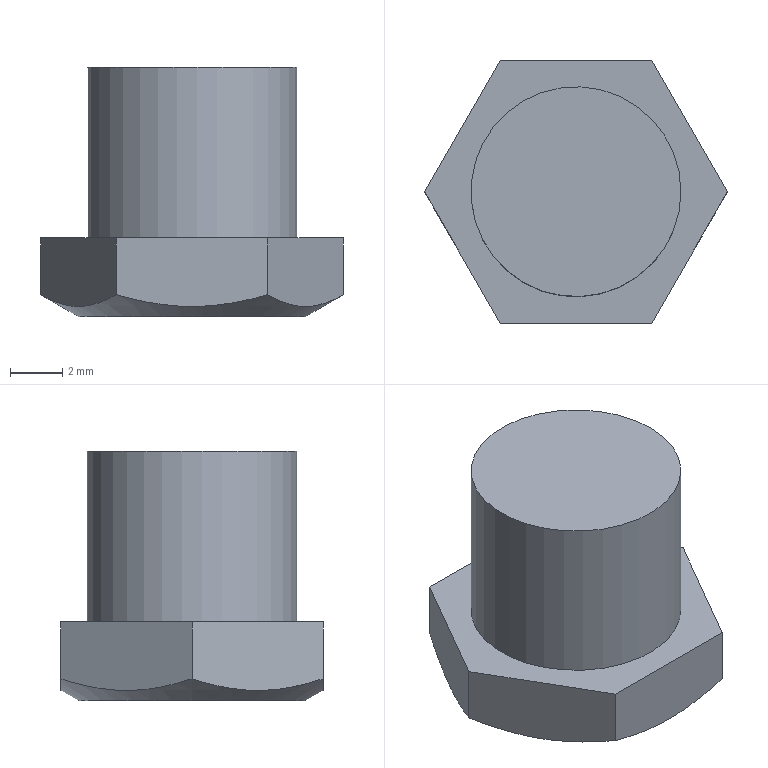Component | NX | BOLT_2 | 1 solid | 11 faces | box 11.55 x 10 x 9.5 mm | volume 578 mm3 | plane 9 | cylinder 1 | cone 1 | commonest cylinder face diameters 8 x1
STEP:
#1=CARTESIAN_POINT('',(0.,0.,0.));
#2=DIRECTION('',(0.,0.,1.));
#3=DIRECTION('',(1.,0.,0.));
#4=AXIS2_PLACEMENT_3D('',#1,#2,#3);
#5=CARTESIAN_POINT('',(-107.5,59.,11.));
#6=VERTEX_POINT('',#5);
#7=CARTESIAN_POINT('',(-111.5,59.,11.));
#8=DIRECTION('',(0.,0.,-1.));
#9=DIRECTION('',(1.,0.,0.));
#10=AXIS2_PLACEMENT_3D('',#7,#8,#9);
#11=CIRCLE('',#10,4.);
#12=CARTESIAN_POINT('',(-111.5,59.,11.));
#13=DIRECTION('',(0.,0.,1.));
#14=DIRECTION('',(-1.,0.,0.));
#15=AXIS2_PLACEMENT_3D('',#12,#13,#14);
#16=PLANE('',#15);
#17=CARTESIAN_POINT('',(-4.,0.));
#18=CARTESIAN_POINT('',(-4.,6.928));
#19=CARTESIAN_POINT('',(2.,3.464));
#20=CARTESIAN_POINT('',(8.,0.));
#21=CARTESIAN_POINT('',(2.,-3.464));
#22=CARTESIAN_POINT('',(-4.,-6.928));
#23=CARTESIAN_POINT('',(-4.,0.));
#24=(BOUNDED_CURVE()B_SPLINE_CURVE(2,(#17,#18,#19,#20,#21,#22,#23),.UNSPECIFIED.,.T.,.F.)B_SPLINE_CURVE_WITH_KNOTS((1,2,2,2,2,1),(-2.094,0.,2.094,4.189,6.283,8.378),.UNSPECIFIED.)CURVE()GEOMETRIC_REPRESENTATION_ITEM()RATIONAL_B_SPLINE_CURVE((1.,0.5,1.,0.5,1.,0.5,1.))REPRESENTATION_ITEM(''));
#25=(GEOMETRIC_REPRESENTATION_CONTEXT(2)PARAMETRIC_REPRESENTATION_CONTEXT()REPRESENTATION_CONTEXT('',''));
#26=DEFINITIONAL_REPRESENTATION('',(#24),#25);
#27=PCURVE('',#16,#26);
#28=CARTESIAN_POINT('',(-111.5,59.,11.));
#29=DIRECTION('',(0.,0.,-1.));
#30=DIRECTION('',(1.,0.,0.));
#31=AXIS2_PLACEMENT_3D('',#28,#29,#30);
#32=CYLINDRICAL_SURFACE('',#31,4.);
#33=CARTESIAN_POINT('',(0.,0.));
#34=DIRECTION('',(1.,0.));
#35=VECTOR('',#34,1.);
#36=LINE('',#33,#35);
#37=(GEOMETRIC_REPRESENTATION_CONTEXT(2)PARAMETRIC_REPRESENTATION_CONTEXT()REPRESENTATION_CONTEXT('',''));
#38=DEFINITIONAL_REPRESENTATION('',(#36),#37);
#39=PCURVE('',#32,#38);
#40=SURFACE_CURVE('',#11,(#27,#39),.PCURVE_S1.);
#41=EDGE_CURVE('',#6,#6,#40,.T.);
#42=ORIENTED_EDGE('',*,*,#41,.F.);
#43=EDGE_LOOP('',(#42));
#44=FACE_BOUND('',#43,.T.);
#45=ADVANCED_FACE('',(#44),#16,.T.);
#46=CARTESIAN_POINT('',(-107.5,59.,4.5));
#47=VERTEX_POINT('',#46);
#48=CARTESIAN_POINT('',(-111.5,59.,4.5));
#49=DIRECTION('',(0.,0.,1.));
#50=DIRECTION('',(1.,0.,0.));
#51=AXIS2_PLACEMENT_3D('',#48,#49,#50);
#52=CIRCLE('',#51,4.);
#53=CARTESIAN_POINT('',(6.283,6.5));
#54=DIRECTION('',(-1.,0.));
#55=VECTOR('',#54,1.);
#56=LINE('',#53,#55);
#57=(GEOMETRIC_REPRESENTATION_CONTEXT(2)PARAMETRIC_REPRESENTATION_CONTEXT()REPRESENTATION_CONTEXT('',''));
#58=DEFINITIONAL_REPRESENTATION('',(#56),#57);
#59=PCURVE('',#32,#58);
#60=CARTESIAN_POINT('',(-111.5,59.,4.5));
#61=DIRECTION('',(0.,0.,1.));
#62=DIRECTION('',(-1.,0.,0.));
#63=AXIS2_PLACEMENT_3D('',#60,#61,#62);
#64=PLANE('',#63);
#65=CARTESIAN_POINT('',(0.,0.));
#66=DIRECTION('',(-1.,0.));
#67=AXIS2_PLACEMENT_2D('',#65,#66);
#68=CIRCLE('',#67,4.);
#69=(GEOMETRIC_REPRESENTATION_CONTEXT(2)PARAMETRIC_REPRESENTATION_CONTEXT()REPRESENTATION_CONTEXT('',''));
#70=DEFINITIONAL_REPRESENTATION('',(#68),#69);
#71=PCURVE('',#64,#70);
#72=SURFACE_CURVE('',#52,(#59,#71),.PCURVE_S1.);
#73=EDGE_CURVE('',#47,#47,#72,.T.);
#74=ORIENTED_EDGE('',*,*,#73,.T.);
#75=CARTESIAN_POINT('',(-107.5,59.,11.));
#76=CARTESIAN_POINT('',(-107.5,59.,4.5));
#77=B_SPLINE_CURVE_WITH_KNOTS('',1,(#75,#76),.UNSPECIFIED.,.F.,.F.,(2,2),(0.,6.5),.PIECEWISE_BEZIER_KNOTS.);
#78=CARTESIAN_POINT('',(0.,0.));
#79=DIRECTION('',(0.,1.));
#80=VECTOR('',#79,1.);
#81=LINE('',#78,#80);
#82=(GEOMETRIC_REPRESENTATION_CONTEXT(2)PARAMETRIC_REPRESENTATION_CONTEXT()REPRESENTATION_CONTEXT('',''));
#83=DEFINITIONAL_REPRESENTATION('',(#81),#82);
#84=PCURVE('',#32,#83);
#85=CARTESIAN_POINT('',(6.283,0.));
#86=DIRECTION('',(0.,1.));
#87=VECTOR('',#86,1.);
#88=LINE('',#85,#87);
#89=(GEOMETRIC_REPRESENTATION_CONTEXT(2)PARAMETRIC_REPRESENTATION_CONTEXT()REPRESENTATION_CONTEXT('',''));
#90=DEFINITIONAL_REPRESENTATION('',(#88),#89);
#91=PCURVE('',#32,#90);
#92=SEAM_CURVE('',#77,(#84,#91),.PCURVE_S1.);
#93=EDGE_CURVE('',#6,#47,#92,.T.);
#94=ORIENTED_EDGE('',*,*,#93,.F.);
#95=ORIENTED_EDGE('',*,*,#41,.T.);
#96=ORIENTED_EDGE('',*,*,#93,.T.);
#97=EDGE_LOOP('',(#74,#94,#95,#96));
#98=FACE_BOUND('',#97,.T.);
#99=ADVANCED_FACE('',(#98),#32,.T.);
#100=CARTESIAN_POINT('',(-105.726,59.,2.333));
#101=VERTEX_POINT('',#100);
#102=CARTESIAN_POINT('',(-108.613,54.,2.333));
#103=VERTEX_POINT('',#102);
#104=CARTESIAN_POINT('',(-105.726,59.,2.333));
#105=CARTESIAN_POINT('',(-106.198,58.184,2.061));
#106=CARTESIAN_POINT('',(-106.676,57.355,1.887));
#107=CARTESIAN_POINT('',(-107.658,55.655,1.886));
#108=CARTESIAN_POINT('',(-108.141,54.817,2.061));
#109=CARTESIAN_POINT('',(-108.613,54.,2.333));
#110=B_SPLINE_CURVE_WITH_KNOTS('',3,(#104,#105,#106,#107,#108,#109),.UNSPECIFIED.,.F.,.F.,(4,2,4),(0.,0.5,1.),.UNSPECIFIED.);
#111=CARTESIAN_POINT('',(-108.613,54.,1.5));
#112=DIRECTION('',(0.866,-0.5,0.));
#113=DIRECTION('',(-0.5,-0.866,0.));
#114=AXIS2_PLACEMENT_3D('',#111,#112,#113);
#115=PLANE('',#114);
#116=CARTESIAN_POINT('',(-5.774,-0.8333));
#117=CARTESIAN_POINT('',(-4.831,-0.5612));
#118=CARTESIAN_POINT('',(-3.874,-0.3874));
#119=CARTESIAN_POINT('',(-1.911,-0.3861));
#120=CARTESIAN_POINT('',(-0.9439,-0.5609));
#121=CARTESIAN_POINT('',(0.,-0.8333));
#122=B_SPLINE_CURVE_WITH_KNOTS('',3,(#116,#117,#118,#119,#120,#121),.UNSPECIFIED.,.F.,.F.,(4,2,4),(0.,0.5,1.),.UNSPECIFIED.);
#123=(GEOMETRIC_REPRESENTATION_CONTEXT(2)PARAMETRIC_REPRESENTATION_CONTEXT()REPRESENTATION_CONTEXT('',''));
#124=DEFINITIONAL_REPRESENTATION('',(#122),#123);
#125=PCURVE('',#115,#124);
#126=CARTESIAN_POINT('',(-111.5,59.,1.5));
#127=DIRECTION('',(0.,0.,1.));
#128=DIRECTION('',(-1.,0.,0.));
#129=AXIS2_PLACEMENT_3D('',#126,#127,#128);
#130=CONICAL_SURFACE('',#129,4.33,1.047);
#131=CARTESIAN_POINT('',(3.142,0.8333));
#132=CARTESIAN_POINT('',(3.129,0.8086));
#133=CARTESIAN_POINT('',(3.102,0.7607));
#134=CARTESIAN_POINT('',(3.061,0.694));
#135=CARTESIAN_POINT('',(3.018,0.6329));
#136=CARTESIAN_POINT('',(2.973,0.5776));
#137=CARTESIAN_POINT('',(2.926,0.5285));
#138=CARTESIAN_POINT('',(2.878,0.4861));
#139=CARTESIAN_POINT('',(2.828,0.4507));
#140=CARTESIAN_POINT('',(2.777,0.4227));
#141=CARTESIAN_POINT('',(2.725,0.4022));
#142=CARTESIAN_POINT('',(2.673,0.3897));
#143=CARTESIAN_POINT('',(2.619,0.3854));
#144=CARTESIAN_POINT('',(2.566,0.3894));
#145=CARTESIAN_POINT('',(2.513,0.4016));
#146=CARTESIAN_POINT('',(2.46,0.4219));
#147=CARTESIAN_POINT('',(2.409,0.4498));
#148=CARTESIAN_POINT('',(2.359,0.4852));
#149=CARTESIAN_POINT('',(2.311,0.5277));
#150=CARTESIAN_POINT('',(2.264,0.5769));
#151=CARTESIAN_POINT('',(2.218,0.6323));
#152=CARTESIAN_POINT('',(2.175,0.6937));
#153=CARTESIAN_POINT('',(2.134,0.7606));
#154=CARTESIAN_POINT('',(2.107,0.8086));
#155=CARTESIAN_POINT('',(2.094,0.8333));
#156=B_SPLINE_CURVE_WITH_KNOTS('',3,(#131,#132,#133,#134,#135,#136,#137,#138,#139,#140,#141,#142,#143,#144,#145,#146,#147,#148,#149,#150,#151,#152,#153,#154,#155),.UNSPECIFIED.,.F.,.F.,(4,1,1,1,1,1,1,1,1,1,1,1,1,1,1,1,1,1,1,1,1,1,4),(0.,0.04545,0.09091,0.1364,0.1818,0.2273,0.2727,0.3182,0.3636,0.4091,0.4545,0.5,0.5455,0.5909,0.6364,0.6818,0.7273,0.7727,0.8182,0.8636,0.9091,0.9545,1.),.QUASI_UNIFORM_KNOTS.);
#157=(GEOMETRIC_REPRESENTATION_CONTEXT(2)PARAMETRIC_REPRESENTATION_CONTEXT()REPRESENTATION_CONTEXT('',''));
#158=DEFINITIONAL_REPRESENTATION('',(#156),#157);
#159=PCURVE('',#130,#158);
#160=SURFACE_CURVE('',#110,(#125,#159),.PCURVE_S1.);
#161=EDGE_CURVE('',#101,#103,#160,.T.);
#162=ORIENTED_EDGE('',*,*,#161,.F.);
#163=CARTESIAN_POINT('',(-105.726,59.,4.5));
#164=VERTEX_POINT('',#163);
#165=CARTESIAN_POINT('',(-105.726,59.,1.5));
#166=DIRECTION('',(0.,0.,1.));
#167=VECTOR('',#166,1.);
#168=LINE('',#165,#167);
#169=CARTESIAN_POINT('',(-5.774,0.));
#170=DIRECTION('',(0.,-1.));
#171=VECTOR('',#170,1.);
#172=LINE('',#169,#171);
#173=(GEOMETRIC_REPRESENTATION_CONTEXT(2)PARAMETRIC_REPRESENTATION_CONTEXT()REPRESENTATION_CONTEXT('',''));
#174=DEFINITIONAL_REPRESENTATION('',(#172),#173);
#175=PCURVE('',#115,#174);
#176=CARTESIAN_POINT('',(-105.726,59.,1.5));
#177=DIRECTION('',(0.866,0.5,0.));
#178=DIRECTION('',(0.5,-0.866,0.));
#179=AXIS2_PLACEMENT_3D('',#176,#177,#178);
#180=PLANE('',#179);
#181=CARTESIAN_POINT('',(0.,0.));
#182=DIRECTION('',(0.,-1.));
#183=VECTOR('',#182,1.);
#184=LINE('',#181,#183);
#185=(GEOMETRIC_REPRESENTATION_CONTEXT(2)PARAMETRIC_REPRESENTATION_CONTEXT()REPRESENTATION_CONTEXT('',''));
#186=DEFINITIONAL_REPRESENTATION('',(#184),#185);
#187=PCURVE('',#180,#186);
#188=SURFACE_CURVE('',#168,(#175,#187),.PCURVE_S1.);
#189=EDGE_CURVE('',#101,#164,#188,.T.);
#190=ORIENTED_EDGE('',*,*,#189,.T.);
#191=CARTESIAN_POINT('',(-108.613,54.,4.5));
#192=VERTEX_POINT('',#191);
#193=CARTESIAN_POINT('',(-108.613,54.,4.5));
#194=DIRECTION('',(0.5,0.866,0.));
#195=VECTOR('',#194,1.);
#196=LINE('',#193,#195);
#197=CARTESIAN_POINT('',(0.,-3.));
#198=DIRECTION('',(-1.,0.));
#199=VECTOR('',#198,1.);
#200=LINE('',#197,#199);
#201=(GEOMETRIC_REPRESENTATION_CONTEXT(2)PARAMETRIC_REPRESENTATION_CONTEXT()REPRESENTATION_CONTEXT('',''));
#202=DEFINITIONAL_REPRESENTATION('',(#200),#201);
#203=PCURVE('',#115,#202);
#204=CARTESIAN_POINT('',(-2.887,5.));
#205=DIRECTION('',(-0.5,-0.866));
#206=VECTOR('',#205,1.);
#207=LINE('',#204,#206);
#208=(GEOMETRIC_REPRESENTATION_CONTEXT(2)PARAMETRIC_REPRESENTATION_CONTEXT()REPRESENTATION_CONTEXT('',''));
#209=DEFINITIONAL_REPRESENTATION('',(#207),#208);
#210=PCURVE('',#64,#209);
#211=SURFACE_CURVE('',#196,(#203,#210),.PCURVE_S1.);
#212=EDGE_CURVE('',#192,#164,#211,.T.);
#213=ORIENTED_EDGE('',*,*,#212,.F.);
#214=CARTESIAN_POINT('',(-108.613,54.,1.5));
#215=DIRECTION('',(0.,0.,1.));
#216=VECTOR('',#215,1.);
#217=LINE('',#214,#216);
#218=CARTESIAN_POINT('',(0.,0.));
#219=DIRECTION('',(0.,-1.));
#220=VECTOR('',#219,1.);
#221=LINE('',#218,#220);
#222=(GEOMETRIC_REPRESENTATION_CONTEXT(2)PARAMETRIC_REPRESENTATION_CONTEXT()REPRESENTATION_CONTEXT('',''));
#223=DEFINITIONAL_REPRESENTATION('',(#221),#222);
#224=PCURVE('',#115,#223);
#225=CARTESIAN_POINT('',(-114.387,54.,1.5));
#226=DIRECTION('',(0.,-1.,0.));
#227=DIRECTION('',(-1.,-0.,0.));
#228=AXIS2_PLACEMENT_3D('',#225,#226,#227);
#229=PLANE('',#228);
#230=CARTESIAN_POINT('',(-5.774,0.));
#231=DIRECTION('',(0.,-1.));
#232=VECTOR('',#231,1.);
#233=LINE('',#230,#232);
#234=(GEOMETRIC_REPRESENTATION_CONTEXT(2)PARAMETRIC_REPRESENTATION_CONTEXT()REPRESENTATION_CONTEXT('',''));
#235=DEFINITIONAL_REPRESENTATION('',(#233),#234);
#236=PCURVE('',#229,#235);
#237=SURFACE_CURVE('',#217,(#224,#236),.PCURVE_S1.);
#238=EDGE_CURVE('',#103,#192,#237,.T.);
#239=ORIENTED_EDGE('',*,*,#238,.F.);
#240=EDGE_LOOP('',(#162,#190,#213,#239));
#241=FACE_BOUND('',#240,.T.);
#242=ADVANCED_FACE('',(#241),#115,.T.);
#243=CARTESIAN_POINT('',(-108.613,64.,2.333));
#244=VERTEX_POINT('',#243);
#245=CARTESIAN_POINT('',(-108.613,64.,2.333));
#246=CARTESIAN_POINT('',(-108.142,63.184,2.061));
#247=CARTESIAN_POINT('',(-107.663,62.355,1.887));
#248=CARTESIAN_POINT('',(-106.682,60.655,1.886));
#249=CARTESIAN_POINT('',(-106.198,59.817,2.061));
#250=CARTESIAN_POINT('',(-105.726,59.,2.333));
#251=B_SPLINE_CURVE_WITH_KNOTS('',3,(#245,#246,#247,#248,#249,#250),.UNSPECIFIED.,.F.,.F.,(4,2,4),(0.,0.5,1.),.UNSPECIFIED.);
#252=CARTESIAN_POINT('',(-5.774,-0.8333));
#253=CARTESIAN_POINT('',(-4.831,-0.5612));
#254=CARTESIAN_POINT('',(-3.874,-0.3874));
#255=CARTESIAN_POINT('',(-1.911,-0.3861));
#256=CARTESIAN_POINT('',(-0.9439,-0.5609));
#257=CARTESIAN_POINT('',(0.,-0.8333));
#258=B_SPLINE_CURVE_WITH_KNOTS('',3,(#252,#253,#254,#255,#256,#257),.UNSPECIFIED.,.F.,.F.,(4,2,4),(0.,0.5,1.),.UNSPECIFIED.);
#259=(GEOMETRIC_REPRESENTATION_CONTEXT(2)PARAMETRIC_REPRESENTATION_CONTEXT()REPRESENTATION_CONTEXT('',''));
#260=DEFINITIONAL_REPRESENTATION('',(#258),#259);
#261=PCURVE('',#180,#260);
#262=CARTESIAN_POINT('',(4.189,0.8333));
#263=CARTESIAN_POINT('',(4.176,0.8086));
#264=CARTESIAN_POINT('',(4.15,0.7607));
#265=CARTESIAN_POINT('',(4.108,0.694));
#266=CARTESIAN_POINT('',(4.065,0.6329));
#267=CARTESIAN_POINT('',(4.02,0.5776));
#268=CARTESIAN_POINT('',(3.974,0.5285));
#269=CARTESIAN_POINT('',(3.925,0.4861));
#270=CARTESIAN_POINT('',(3.876,0.4507));
#271=CARTESIAN_POINT('',(3.825,0.4227));
#272=CARTESIAN_POINT('',(3.773,0.4022));
#273=CARTESIAN_POINT('',(3.72,0.3897));
#274=CARTESIAN_POINT('',(3.666,0.3854));
#275=CARTESIAN_POINT('',(3.613,0.3894));
#276=CARTESIAN_POINT('',(3.56,0.4016));
#277=CARTESIAN_POINT('',(3.507,0.4219));
#278=CARTESIAN_POINT('',(3.456,0.4498));
#279=CARTESIAN_POINT('',(3.406,0.4852));
#280=CARTESIAN_POINT('',(3.358,0.5277));
#281=CARTESIAN_POINT('',(3.311,0.5769));
#282=CARTESIAN_POINT('',(3.266,0.6323));
#283=CARTESIAN_POINT('',(3.222,0.6937));
#284=CARTESIAN_POINT('',(3.181,0.7606));
#285=CARTESIAN_POINT('',(3.154,0.8086));
#286=CARTESIAN_POINT('',(3.142,0.8333));
#287=B_SPLINE_CURVE_WITH_KNOTS('',3,(#262,#263,#264,#265,#266,#267,#268,#269,#270,#271,#272,#273,#274,#275,#276,#277,#278,#279,#280,#281,#282,#283,#284,#285,#286),.UNSPECIFIED.,.F.,.F.,(4,1,1,1,1,1,1,1,1,1,1,1,1,1,1,1,1,1,1,1,1,1,4),(0.,0.04545,0.09091,0.1364,0.1818,0.2273,0.2727,0.3182,0.3636,0.4091,0.4545,0.5,0.5455,0.5909,0.6364,0.6818,0.7273,0.7727,0.8182,0.8636,0.9091,0.9545,1.),.QUASI_UNIFORM_KNOTS.);
#288=(GEOMETRIC_REPRESENTATION_CONTEXT(2)PARAMETRIC_REPRESENTATION_CONTEXT()REPRESENTATION_CONTEXT('',''));
#289=DEFINITIONAL_REPRESENTATION('',(#287),#288);
#290=PCURVE('',#130,#289);
#291=SURFACE_CURVE('',#251,(#261,#290),.PCURVE_S1.);
#292=EDGE_CURVE('',#244,#101,#291,.T.);
#293=ORIENTED_EDGE('',*,*,#292,.F.);
#294=CARTESIAN_POINT('',(-108.613,64.,4.5));
#295=VERTEX_POINT('',#294);
#296=CARTESIAN_POINT('',(-108.613,64.,1.5));
#297=DIRECTION('',(0.,0.,1.));
#298=VECTOR('',#297,1.);
#299=LINE('',#296,#298);
#300=CARTESIAN_POINT('',(-5.774,0.));
#301=DIRECTION('',(0.,-1.));
#302=VECTOR('',#301,1.);
#303=LINE('',#300,#302);
#304=(GEOMETRIC_REPRESENTATION_CONTEXT(2)PARAMETRIC_REPRESENTATION_CONTEXT()REPRESENTATION_CONTEXT('',''));
#305=DEFINITIONAL_REPRESENTATION('',(#303),#304);
#306=PCURVE('',#180,#305);
#307=CARTESIAN_POINT('',(-108.613,64.,1.5));
#308=DIRECTION('',(-0.,1.,0.));
#309=DIRECTION('',(1.,0.,0.));
#310=AXIS2_PLACEMENT_3D('',#307,#308,#309);
#311=PLANE('',#310);
#312=CARTESIAN_POINT('',(0.,0.));
#313=DIRECTION('',(0.,-1.));
#314=VECTOR('',#313,1.);
#315=LINE('',#312,#314);
#316=(GEOMETRIC_REPRESENTATION_CONTEXT(2)PARAMETRIC_REPRESENTATION_CONTEXT()REPRESENTATION_CONTEXT('',''));
#317=DEFINITIONAL_REPRESENTATION('',(#315),#316);
#318=PCURVE('',#311,#317);
#319=SURFACE_CURVE('',#299,(#306,#318),.PCURVE_S1.);
#320=EDGE_CURVE('',#244,#295,#319,.T.);
#321=ORIENTED_EDGE('',*,*,#320,.T.);
#322=CARTESIAN_POINT('',(-105.726,59.,4.5));
#323=DIRECTION('',(-0.5,0.866,0.));
#324=VECTOR('',#323,1.);
#325=LINE('',#322,#324);
#326=CARTESIAN_POINT('',(0.,-3.));
#327=DIRECTION('',(-1.,0.));
#328=VECTOR('',#327,1.);
#329=LINE('',#326,#328);
#330=(GEOMETRIC_REPRESENTATION_CONTEXT(2)PARAMETRIC_REPRESENTATION_CONTEXT()REPRESENTATION_CONTEXT('',''));
#331=DEFINITIONAL_REPRESENTATION('',(#329),#330);
#332=PCURVE('',#180,#331);
#333=CARTESIAN_POINT('',(-5.774,0.));
#334=DIRECTION('',(0.5,-0.866));
#335=VECTOR('',#334,1.);
#336=LINE('',#333,#335);
#337=(GEOMETRIC_REPRESENTATION_CONTEXT(2)PARAMETRIC_REPRESENTATION_CONTEXT()REPRESENTATION_CONTEXT('',''));
#338=DEFINITIONAL_REPRESENTATION('',(#336),#337);
#339=PCURVE('',#64,#338);
#340=SURFACE_CURVE('',#325,(#332,#339),.PCURVE_S1.);
#341=EDGE_CURVE('',#164,#295,#340,.T.);
#342=ORIENTED_EDGE('',*,*,#341,.F.);
#343=ORIENTED_EDGE('',*,*,#189,.F.);
#344=EDGE_LOOP('',(#293,#321,#342,#343));
#345=FACE_BOUND('',#344,.T.);
#346=ADVANCED_FACE('',(#345),#180,.T.);
#347=CARTESIAN_POINT('',(-114.387,64.,2.333));
#348=VERTEX_POINT('',#347);
#349=CARTESIAN_POINT('',(-114.387,64.,2.333));
#350=CARTESIAN_POINT('',(-113.448,64.,2.062));
#351=CARTESIAN_POINT('',(-112.475,64.,1.887));
#352=CARTESIAN_POINT('',(-110.524,64.,1.887));
#353=CARTESIAN_POINT('',(-109.546,64.,2.064));
#354=CARTESIAN_POINT('',(-108.613,64.,2.333));
#355=B_SPLINE_CURVE_WITH_KNOTS('',3,(#349,#350,#351,#352,#353,#354),.UNSPECIFIED.,.F.,.F.,(4,2,4),(0.,0.5,1.),.UNSPECIFIED.);
#356=CARTESIAN_POINT('',(-5.774,-0.8333));
#357=CARTESIAN_POINT('',(-4.835,-0.5623));
#358=CARTESIAN_POINT('',(-3.862,-0.3867));
#359=CARTESIAN_POINT('',(-1.91,-0.3868));
#360=CARTESIAN_POINT('',(-0.9332,-0.5639));
#361=CARTESIAN_POINT('',(0.,-0.8333));
#362=B_SPLINE_CURVE_WITH_KNOTS('',3,(#356,#357,#358,#359,#360,#361),.UNSPECIFIED.,.F.,.F.,(4,2,4),(0.,0.5,1.),.UNSPECIFIED.);
#363=(GEOMETRIC_REPRESENTATION_CONTEXT(2)PARAMETRIC_REPRESENTATION_CONTEXT()REPRESENTATION_CONTEXT('',''));
#364=DEFINITIONAL_REPRESENTATION('',(#362),#363);
#365=PCURVE('',#311,#364);
#366=CARTESIAN_POINT('',(5.236,0.8333));
#367=CARTESIAN_POINT('',(5.223,0.8087));
#368=CARTESIAN_POINT('',(5.197,0.7609));
#369=CARTESIAN_POINT('',(5.156,0.6942));
#370=CARTESIAN_POINT('',(5.112,0.6329));
#371=CARTESIAN_POINT('',(5.067,0.5774));
#372=CARTESIAN_POINT('',(5.02,0.5282));
#373=CARTESIAN_POINT('',(4.972,0.4856));
#374=CARTESIAN_POINT('',(4.922,0.4502));
#375=CARTESIAN_POINT('',(4.87,0.4221));
#376=CARTESIAN_POINT('',(4.818,0.4018));
#377=CARTESIAN_POINT('',(4.765,0.3895));
#378=CARTESIAN_POINT('',(4.712,0.3854));
#379=CARTESIAN_POINT('',(4.659,0.3896));
#380=CARTESIAN_POINT('',(4.606,0.4019));
#381=CARTESIAN_POINT('',(4.554,0.4224));
#382=CARTESIAN_POINT('',(4.503,0.4505));
#383=CARTESIAN_POINT('',(4.453,0.4861));
#384=CARTESIAN_POINT('',(4.404,0.5287));
#385=CARTESIAN_POINT('',(4.357,0.578));
#386=CARTESIAN_POINT('',(4.312,0.6335));
#387=CARTESIAN_POINT('',(4.269,0.6948));
#388=CARTESIAN_POINT('',(4.228,0.7613));
#389=CARTESIAN_POINT('',(4.202,0.8088));
#390=CARTESIAN_POINT('',(4.189,0.8333));
#391=B_SPLINE_CURVE_WITH_KNOTS('',3,(#366,#367,#368,#369,#370,#371,#372,#373,#374,#375,#376,#377,#378,#379,#380,#381,#382,#383,#384,#385,#386,#387,#388,#389,#390),.UNSPECIFIED.,.F.,.F.,(4,1,1,1,1,1,1,1,1,1,1,1,1,1,1,1,1,1,1,1,1,1,4),(0.,0.04545,0.09091,0.1364,0.1818,0.2273,0.2727,0.3182,0.3636,0.4091,0.4545,0.5,0.5455,0.5909,0.6364,0.6818,0.7273,0.7727,0.8182,0.8636,0.9091,0.9545,1.),.QUASI_UNIFORM_KNOTS.);
#392=(GEOMETRIC_REPRESENTATION_CONTEXT(2)PARAMETRIC_REPRESENTATION_CONTEXT()REPRESENTATION_CONTEXT('',''));
#393=DEFINITIONAL_REPRESENTATION('',(#391),#392);
#394=PCURVE('',#130,#393);
#395=SURFACE_CURVE('',#355,(#365,#394),.PCURVE_S1.);
#396=EDGE_CURVE('',#348,#244,#395,.T.);
#397=ORIENTED_EDGE('',*,*,#396,.F.);
#398=CARTESIAN_POINT('',(-114.387,64.,4.5));
#399=VERTEX_POINT('',#398);
#400=CARTESIAN_POINT('',(-114.387,64.,1.5));
#401=DIRECTION('',(0.,0.,1.));
#402=VECTOR('',#401,1.);
#403=LINE('',#400,#402);
#404=CARTESIAN_POINT('',(-5.774,0.));
#405=DIRECTION('',(0.,-1.));
#406=VECTOR('',#405,1.);
#407=LINE('',#404,#406);
#408=(GEOMETRIC_REPRESENTATION_CONTEXT(2)PARAMETRIC_REPRESENTATION_CONTEXT()REPRESENTATION_CONTEXT('',''));
#409=DEFINITIONAL_REPRESENTATION('',(#407),#408);
#410=PCURVE('',#311,#409);
#411=CARTESIAN_POINT('',(-114.387,64.,1.5));
#412=DIRECTION('',(-0.866,0.5,0.));
#413=DIRECTION('',(0.5,0.866,0.));
#414=AXIS2_PLACEMENT_3D('',#411,#412,#413);
#415=PLANE('',#414);
#416=CARTESIAN_POINT('',(0.,0.));
#417=DIRECTION('',(0.,-1.));
#418=VECTOR('',#417,1.);
#419=LINE('',#416,#418);
#420=(GEOMETRIC_REPRESENTATION_CONTEXT(2)PARAMETRIC_REPRESENTATION_CONTEXT()REPRESENTATION_CONTEXT('',''));
#421=DEFINITIONAL_REPRESENTATION('',(#419),#420);
#422=PCURVE('',#415,#421);
#423=SURFACE_CURVE('',#403,(#410,#422),.PCURVE_S1.);
#424=EDGE_CURVE('',#348,#399,#423,.T.);
#425=ORIENTED_EDGE('',*,*,#424,.T.);
#426=CARTESIAN_POINT('',(-108.613,64.,4.5));
#427=DIRECTION('',(-1.,-0.,0.));
#428=VECTOR('',#427,1.);
#429=LINE('',#426,#428);
#430=CARTESIAN_POINT('',(0.,-3.));
#431=DIRECTION('',(-1.,0.));
#432=VECTOR('',#431,1.);
#433=LINE('',#430,#432);
#434=(GEOMETRIC_REPRESENTATION_CONTEXT(2)PARAMETRIC_REPRESENTATION_CONTEXT()REPRESENTATION_CONTEXT('',''));
#435=DEFINITIONAL_REPRESENTATION('',(#433),#434);
#436=PCURVE('',#311,#435);
#437=CARTESIAN_POINT('',(-2.887,-5.));
#438=DIRECTION('',(1.,0.));
#439=VECTOR('',#438,1.);
#440=LINE('',#437,#439);
#441=(GEOMETRIC_REPRESENTATION_CONTEXT(2)PARAMETRIC_REPRESENTATION_CONTEXT()REPRESENTATION_CONTEXT('',''));
#442=DEFINITIONAL_REPRESENTATION('',(#440),#441);
#443=PCURVE('',#64,#442);
#444=SURFACE_CURVE('',#429,(#436,#443),.PCURVE_S1.);
#445=EDGE_CURVE('',#295,#399,#444,.T.);
#446=ORIENTED_EDGE('',*,*,#445,.F.);
#447=ORIENTED_EDGE('',*,*,#320,.F.);
#448=EDGE_LOOP('',(#397,#425,#446,#447));
#449=FACE_BOUND('',#448,.T.);
#450=ADVANCED_FACE('',(#449),#311,.T.);
#451=CARTESIAN_POINT('',(-117.274,59.,2.333));
#452=VERTEX_POINT('',#451);
#453=CARTESIAN_POINT('',(-117.274,59.,2.333));
#454=CARTESIAN_POINT('',(-116.802,59.816,2.061));
#455=CARTESIAN_POINT('',(-116.324,60.645,1.887));
#456=CARTESIAN_POINT('',(-115.342,62.345,1.886));
#457=CARTESIAN_POINT('',(-114.859,63.183,2.061));
#458=CARTESIAN_POINT('',(-114.387,64.,2.333));
#459=B_SPLINE_CURVE_WITH_KNOTS('',3,(#453,#454,#455,#456,#457,#458),.UNSPECIFIED.,.F.,.F.,(4,2,4),(0.,0.5,1.),.UNSPECIFIED.);
#460=CARTESIAN_POINT('',(-5.774,-0.8333));
#461=CARTESIAN_POINT('',(-4.831,-0.5612));
#462=CARTESIAN_POINT('',(-3.874,-0.3874));
#463=CARTESIAN_POINT('',(-1.911,-0.3861));
#464=CARTESIAN_POINT('',(-0.9439,-0.5609));
#465=CARTESIAN_POINT('',(0.,-0.8333));
#466=B_SPLINE_CURVE_WITH_KNOTS('',3,(#460,#461,#462,#463,#464,#465),.UNSPECIFIED.,.F.,.F.,(4,2,4),(0.,0.5,1.),.UNSPECIFIED.);
#467=(GEOMETRIC_REPRESENTATION_CONTEXT(2)PARAMETRIC_REPRESENTATION_CONTEXT()REPRESENTATION_CONTEXT('',''));
#468=DEFINITIONAL_REPRESENTATION('',(#466),#467);
#469=PCURVE('',#415,#468);
#470=CARTESIAN_POINT('',(6.283,0.8333));
#471=CARTESIAN_POINT('',(6.27,0.8086));
#472=CARTESIAN_POINT('',(6.244,0.7607));
#473=CARTESIAN_POINT('',(6.203,0.694));
#474=CARTESIAN_POINT('',(6.16,0.6329));
#475=CARTESIAN_POINT('',(6.115,0.5776));
#476=CARTESIAN_POINT('',(6.068,0.5285));
#477=CARTESIAN_POINT('',(6.02,0.4861));
#478=CARTESIAN_POINT('',(5.97,0.4507));
#479=CARTESIAN_POINT('',(5.919,0.4227));
#480=CARTESIAN_POINT('',(5.867,0.4022));
#481=CARTESIAN_POINT('',(5.814,0.3897));
#482=CARTESIAN_POINT('',(5.761,0.3854));
#483=CARTESIAN_POINT('',(5.707,0.3894));
#484=CARTESIAN_POINT('',(5.654,0.4016));
#485=CARTESIAN_POINT('',(5.602,0.4219));
#486=CARTESIAN_POINT('',(5.551,0.4498));
#487=CARTESIAN_POINT('',(5.501,0.4852));
#488=CARTESIAN_POINT('',(5.452,0.5277));
#489=CARTESIAN_POINT('',(5.405,0.5769));
#490=CARTESIAN_POINT('',(5.36,0.6323));
#491=CARTESIAN_POINT('',(5.317,0.6937));
#492=CARTESIAN_POINT('',(5.275,0.7606));
#493=CARTESIAN_POINT('',(5.249,0.8086));
#494=CARTESIAN_POINT('',(5.236,0.8333));
#495=B_SPLINE_CURVE_WITH_KNOTS('',3,(#470,#471,#472,#473,#474,#475,#476,#477,#478,#479,#480,#481,#482,#483,#484,#485,#486,#487,#488,#489,#490,#491,#492,#493,#494),.UNSPECIFIED.,.F.,.F.,(4,1,1,1,1,1,1,1,1,1,1,1,1,1,1,1,1,1,1,1,1,1,4),(0.,0.04545,0.09091,0.1364,0.1818,0.2273,0.2727,0.3182,0.3636,0.4091,0.4545,0.5,0.5455,0.5909,0.6364,0.6818,0.7273,0.7727,0.8182,0.8636,0.9091,0.9545,1.),.QUASI_UNIFORM_KNOTS.);
#496=(GEOMETRIC_REPRESENTATION_CONTEXT(2)PARAMETRIC_REPRESENTATION_CONTEXT()REPRESENTATION_CONTEXT('',''));
#497=DEFINITIONAL_REPRESENTATION('',(#495),#496);
#498=PCURVE('',#130,#497);
#499=SURFACE_CURVE('',#459,(#469,#498),.PCURVE_S1.);
#500=EDGE_CURVE('',#452,#348,#499,.T.);
#501=ORIENTED_EDGE('',*,*,#500,.F.);
#502=CARTESIAN_POINT('',(-117.274,59.,4.5));
#503=VERTEX_POINT('',#502);
#504=CARTESIAN_POINT('',(-117.274,59.,1.5));
#505=DIRECTION('',(0.,0.,1.));
#506=VECTOR('',#505,1.);
#507=LINE('',#504,#506);
#508=CARTESIAN_POINT('',(-5.774,0.));
#509=DIRECTION('',(0.,-1.));
#510=VECTOR('',#509,1.);
#511=LINE('',#508,#510);
#512=(GEOMETRIC_REPRESENTATION_CONTEXT(2)PARAMETRIC_REPRESENTATION_CONTEXT()REPRESENTATION_CONTEXT('',''));
#513=DEFINITIONAL_REPRESENTATION('',(#511),#512);
#514=PCURVE('',#415,#513);
#515=CARTESIAN_POINT('',(-117.274,59.,1.5));
#516=DIRECTION('',(-0.866,-0.5,0.));
#517=DIRECTION('',(-0.5,0.866,0.));
#518=AXIS2_PLACEMENT_3D('',#515,#516,#517);
#519=PLANE('',#518);
#520=CARTESIAN_POINT('',(0.,0.));
#521=DIRECTION('',(0.,-1.));
#522=VECTOR('',#521,1.);
#523=LINE('',#520,#522);
#524=(GEOMETRIC_REPRESENTATION_CONTEXT(2)PARAMETRIC_REPRESENTATION_CONTEXT()REPRESENTATION_CONTEXT('',''));
#525=DEFINITIONAL_REPRESENTATION('',(#523),#524);
#526=PCURVE('',#519,#525);
#527=SURFACE_CURVE('',#507,(#514,#526),.PCURVE_S1.);
#528=EDGE_CURVE('',#452,#503,#527,.T.);
#529=ORIENTED_EDGE('',*,*,#528,.T.);
#530=CARTESIAN_POINT('',(-114.387,64.,4.5));
#531=DIRECTION('',(-0.5,-0.866,0.));
#532=VECTOR('',#531,1.);
#533=LINE('',#530,#532);
#534=CARTESIAN_POINT('',(0.,-3.));
#535=DIRECTION('',(-1.,0.));
#536=VECTOR('',#535,1.);
#537=LINE('',#534,#536);
#538=(GEOMETRIC_REPRESENTATION_CONTEXT(2)PARAMETRIC_REPRESENTATION_CONTEXT()REPRESENTATION_CONTEXT('',''));
#539=DEFINITIONAL_REPRESENTATION('',(#537),#538);
#540=PCURVE('',#415,#539);
#541=CARTESIAN_POINT('',(2.887,-5.));
#542=DIRECTION('',(0.5,0.866));
#543=VECTOR('',#542,1.);
#544=LINE('',#541,#543);
#545=(GEOMETRIC_REPRESENTATION_CONTEXT(2)PARAMETRIC_REPRESENTATION_CONTEXT()REPRESENTATION_CONTEXT('',''));
#546=DEFINITIONAL_REPRESENTATION('',(#544),#545);
#547=PCURVE('',#64,#546);
#548=SURFACE_CURVE('',#533,(#540,#547),.PCURVE_S1.);
#549=EDGE_CURVE('',#399,#503,#548,.T.);
#550=ORIENTED_EDGE('',*,*,#549,.F.);
#551=ORIENTED_EDGE('',*,*,#424,.F.);
#552=EDGE_LOOP('',(#501,#529,#550,#551));
#553=FACE_BOUND('',#552,.T.);
#554=ADVANCED_FACE('',(#553),#415,.T.);
#555=CARTESIAN_POINT('',(-114.387,54.,2.333));
#556=VERTEX_POINT('',#555);
#557=CARTESIAN_POINT('',(-114.387,54.,2.333));
#558=CARTESIAN_POINT('',(-114.858,54.816,2.061));
#559=CARTESIAN_POINT('',(-115.337,55.645,1.887));
#560=CARTESIAN_POINT('',(-116.318,57.345,1.886));
#561=CARTESIAN_POINT('',(-116.802,58.183,2.061));
#562=CARTESIAN_POINT('',(-117.274,59.,2.333));
#563=B_SPLINE_CURVE_WITH_KNOTS('',3,(#557,#558,#559,#560,#561,#562),.UNSPECIFIED.,.F.,.F.,(4,2,4),(0.,0.5,1.),.UNSPECIFIED.);
#564=CARTESIAN_POINT('',(-5.774,-0.8333));
#565=CARTESIAN_POINT('',(-4.831,-0.5612));
#566=CARTESIAN_POINT('',(-3.874,-0.3874));
#567=CARTESIAN_POINT('',(-1.911,-0.3861));
#568=CARTESIAN_POINT('',(-0.9439,-0.5609));
#569=CARTESIAN_POINT('',(0.,-0.8333));
#570=B_SPLINE_CURVE_WITH_KNOTS('',3,(#564,#565,#566,#567,#568,#569),.UNSPECIFIED.,.F.,.F.,(4,2,4),(0.,0.5,1.),.UNSPECIFIED.);
#571=(GEOMETRIC_REPRESENTATION_CONTEXT(2)PARAMETRIC_REPRESENTATION_CONTEXT()REPRESENTATION_CONTEXT('',''));
#572=DEFINITIONAL_REPRESENTATION('',(#570),#571);
#573=PCURVE('',#519,#572);
#574=CARTESIAN_POINT('',(1.047,0.8333));
#575=CARTESIAN_POINT('',(1.034,0.8086));
#576=CARTESIAN_POINT('',(1.008,0.7607));
#577=CARTESIAN_POINT('',(0.9667,0.694));
#578=CARTESIAN_POINT('',(0.9236,0.6329));
#579=CARTESIAN_POINT('',(0.8787,0.5776));
#580=CARTESIAN_POINT('',(0.832,0.5285));
#581=CARTESIAN_POINT('',(0.7838,0.4861));
#582=CARTESIAN_POINT('',(0.7341,0.4507));
#583=CARTESIAN_POINT('',(0.6831,0.4227));
#584=CARTESIAN_POINT('',(0.631,0.4022));
#585=CARTESIAN_POINT('',(0.5782,0.3897));
#586=CARTESIAN_POINT('',(0.5247,0.3854));
#587=CARTESIAN_POINT('',(0.4712,0.3894));
#588=CARTESIAN_POINT('',(0.4182,0.4016));
#589=CARTESIAN_POINT('',(0.3659,0.4219));
#590=CARTESIAN_POINT('',(0.3147,0.4498));
#591=CARTESIAN_POINT('',(0.2647,0.4852));
#592=CARTESIAN_POINT('',(0.2161,0.5277));
#593=CARTESIAN_POINT('',(0.1692,0.5769));
#594=CARTESIAN_POINT('',(0.124,0.6323));
#595=CARTESIAN_POINT('',(0.0807,0.6937));
#596=CARTESIAN_POINT('',(0.03925,0.7606));
#597=CARTESIAN_POINT('',(0.01287,0.8086));
#598=CARTESIAN_POINT('',(0.,0.8333));
#599=B_SPLINE_CURVE_WITH_KNOTS('',3,(#574,#575,#576,#577,#578,#579,#580,#581,#582,#583,#584,#585,#586,#587,#588,#589,#590,#591,#592,#593,#594,#595,#596,#597,#598),.UNSPECIFIED.,.F.,.F.,(4,1,1,1,1,1,1,1,1,1,1,1,1,1,1,1,1,1,1,1,1,1,4),(0.,0.04545,0.09091,0.1364,0.1818,0.2273,0.2727,0.3182,0.3636,0.4091,0.4545,0.5,0.5455,0.5909,0.6364,0.6818,0.7273,0.7727,0.8182,0.8636,0.9091,0.9545,1.),.QUASI_UNIFORM_KNOTS.);
#600=(GEOMETRIC_REPRESENTATION_CONTEXT(2)PARAMETRIC_REPRESENTATION_CONTEXT()REPRESENTATION_CONTEXT('',''));
#601=DEFINITIONAL_REPRESENTATION('',(#599),#600);
#602=PCURVE('',#130,#601);
#603=SURFACE_CURVE('',#563,(#573,#602),.PCURVE_S1.);
#604=EDGE_CURVE('',#556,#452,#603,.T.);
#605=ORIENTED_EDGE('',*,*,#604,.F.);
#606=CARTESIAN_POINT('',(-114.387,54.,4.5));
#607=VERTEX_POINT('',#606);
#608=CARTESIAN_POINT('',(-114.387,54.,1.5));
#609=DIRECTION('',(0.,0.,1.));
#610=VECTOR('',#609,1.);
#611=LINE('',#608,#610);
#612=CARTESIAN_POINT('',(-5.774,0.));
#613=DIRECTION('',(0.,-1.));
#614=VECTOR('',#613,1.);
#615=LINE('',#612,#614);
#616=(GEOMETRIC_REPRESENTATION_CONTEXT(2)PARAMETRIC_REPRESENTATION_CONTEXT()REPRESENTATION_CONTEXT('',''));
#617=DEFINITIONAL_REPRESENTATION('',(#615),#616);
#618=PCURVE('',#519,#617);
#619=CARTESIAN_POINT('',(0.,0.));
#620=DIRECTION('',(0.,-1.));
#621=VECTOR('',#620,1.);
#622=LINE('',#619,#621);
#623=(GEOMETRIC_REPRESENTATION_CONTEXT(2)PARAMETRIC_REPRESENTATION_CONTEXT()REPRESENTATION_CONTEXT('',''));
#624=DEFINITIONAL_REPRESENTATION('',(#622),#623);
#625=PCURVE('',#229,#624);
#626=SURFACE_CURVE('',#611,(#618,#625),.PCURVE_S1.);
#627=EDGE_CURVE('',#556,#607,#626,.T.);
#628=ORIENTED_EDGE('',*,*,#627,.T.);
#629=CARTESIAN_POINT('',(-117.274,59.,4.5));
#630=DIRECTION('',(0.5,-0.866,0.));
#631=VECTOR('',#630,1.);
#632=LINE('',#629,#631);
#633=CARTESIAN_POINT('',(0.,-3.));
#634=DIRECTION('',(-1.,0.));
#635=VECTOR('',#634,1.);
#636=LINE('',#633,#635);
#637=(GEOMETRIC_REPRESENTATION_CONTEXT(2)PARAMETRIC_REPRESENTATION_CONTEXT()REPRESENTATION_CONTEXT('',''));
#638=DEFINITIONAL_REPRESENTATION('',(#636),#637);
#639=PCURVE('',#519,#638);
#640=CARTESIAN_POINT('',(5.774,0.));
#641=DIRECTION('',(-0.5,0.866));
#642=VECTOR('',#641,1.);
#643=LINE('',#640,#642);
#644=(GEOMETRIC_REPRESENTATION_CONTEXT(2)PARAMETRIC_REPRESENTATION_CONTEXT()REPRESENTATION_CONTEXT('',''));
#645=DEFINITIONAL_REPRESENTATION('',(#643),#644);
#646=PCURVE('',#64,#645);
#647=SURFACE_CURVE('',#632,(#639,#646),.PCURVE_S1.);
#648=EDGE_CURVE('',#503,#607,#647,.T.);
#649=ORIENTED_EDGE('',*,*,#648,.F.);
#650=ORIENTED_EDGE('',*,*,#528,.F.);
#651=EDGE_LOOP('',(#605,#628,#649,#650));
#652=FACE_BOUND('',#651,.T.);
#653=ADVANCED_FACE('',(#652),#519,.T.);
#654=CARTESIAN_POINT('',(-108.613,54.,2.333));
#655=CARTESIAN_POINT('',(-109.546,54.,2.064));
#656=CARTESIAN_POINT('',(-110.524,54.,1.887));
#657=CARTESIAN_POINT('',(-112.475,54.,1.887));
#658=CARTESIAN_POINT('',(-113.448,54.,2.062));
#659=CARTESIAN_POINT('',(-114.387,54.,2.333));
#660=B_SPLINE_CURVE_WITH_KNOTS('',3,(#654,#655,#656,#657,#658,#659),.UNSPECIFIED.,.F.,.F.,(4,2,4),(0.,0.5,1.),.UNSPECIFIED.);
#661=CARTESIAN_POINT('',(-5.774,-0.8333));
#662=CARTESIAN_POINT('',(-4.84,-0.5639));
#663=CARTESIAN_POINT('',(-3.863,-0.3868));
#664=CARTESIAN_POINT('',(-1.912,-0.3867));
#665=CARTESIAN_POINT('',(-0.9389,-0.5623));
#666=CARTESIAN_POINT('',(0.,-0.8333));
#667=B_SPLINE_CURVE_WITH_KNOTS('',3,(#661,#662,#663,#664,#665,#666),.UNSPECIFIED.,.F.,.F.,(4,2,4),(0.,0.5,1.),.UNSPECIFIED.);
#668=(GEOMETRIC_REPRESENTATION_CONTEXT(2)PARAMETRIC_REPRESENTATION_CONTEXT()REPRESENTATION_CONTEXT('',''));
#669=DEFINITIONAL_REPRESENTATION('',(#667),#668);
#670=PCURVE('',#229,#669);
#671=CARTESIAN_POINT('',(2.094,0.8333));
#672=CARTESIAN_POINT('',(2.082,0.8088));
#673=CARTESIAN_POINT('',(2.056,0.7613));
#674=CARTESIAN_POINT('',(2.014,0.6948));
#675=CARTESIAN_POINT('',(1.971,0.6335));
#676=CARTESIAN_POINT('',(1.926,0.578));
#677=CARTESIAN_POINT('',(1.879,0.5287));
#678=CARTESIAN_POINT('',(1.831,0.4861));
#679=CARTESIAN_POINT('',(1.781,0.4505));
#680=CARTESIAN_POINT('',(1.729,0.4224));
#681=CARTESIAN_POINT('',(1.677,0.4019));
#682=CARTESIAN_POINT('',(1.624,0.3896));
#683=CARTESIAN_POINT('',(1.571,0.3854));
#684=CARTESIAN_POINT('',(1.518,0.3895));
#685=CARTESIAN_POINT('',(1.465,0.4018));
#686=CARTESIAN_POINT('',(1.413,0.4221));
#687=CARTESIAN_POINT('',(1.362,0.4502));
#688=CARTESIAN_POINT('',(1.312,0.4856));
#689=CARTESIAN_POINT('',(1.263,0.5282));
#690=CARTESIAN_POINT('',(1.216,0.5774));
#691=CARTESIAN_POINT('',(1.171,0.6329));
#692=CARTESIAN_POINT('',(1.128,0.6942));
#693=CARTESIAN_POINT('',(1.086,0.7609));
#694=CARTESIAN_POINT('',(1.06,0.8087));
#695=CARTESIAN_POINT('',(1.047,0.8333));
#696=B_SPLINE_CURVE_WITH_KNOTS('',3,(#671,#672,#673,#674,#675,#676,#677,#678,#679,#680,#681,#682,#683,#684,#685,#686,#687,#688,#689,#690,#691,#692,#693,#694,#695),.UNSPECIFIED.,.F.,.F.,(4,1,1,1,1,1,1,1,1,1,1,1,1,1,1,1,1,1,1,1,1,1,4),(0.,0.04545,0.09091,0.1364,0.1818,0.2273,0.2727,0.3182,0.3636,0.4091,0.4545,0.5,0.5455,0.5909,0.6364,0.6818,0.7273,0.7727,0.8182,0.8636,0.9091,0.9545,1.),.QUASI_UNIFORM_KNOTS.);
#697=(GEOMETRIC_REPRESENTATION_CONTEXT(2)PARAMETRIC_REPRESENTATION_CONTEXT()REPRESENTATION_CONTEXT('',''));
#698=DEFINITIONAL_REPRESENTATION('',(#696),#697);
#699=PCURVE('',#130,#698);
#700=SURFACE_CURVE('',#660,(#670,#699),.PCURVE_S1.);
#701=EDGE_CURVE('',#103,#556,#700,.T.);
#702=ORIENTED_EDGE('',*,*,#701,.F.);
#703=ORIENTED_EDGE('',*,*,#238,.T.);
#704=CARTESIAN_POINT('',(-114.387,54.,4.5));
#705=DIRECTION('',(1.,0.,0.));
#706=VECTOR('',#705,1.);
#707=LINE('',#704,#706);
#708=CARTESIAN_POINT('',(0.,-3.));
#709=DIRECTION('',(-1.,0.));
#710=VECTOR('',#709,1.);
#711=LINE('',#708,#710);
#712=(GEOMETRIC_REPRESENTATION_CONTEXT(2)PARAMETRIC_REPRESENTATION_CONTEXT()REPRESENTATION_CONTEXT('',''));
#713=DEFINITIONAL_REPRESENTATION('',(#711),#712);
#714=PCURVE('',#229,#713);
#715=CARTESIAN_POINT('',(2.887,5.));
#716=DIRECTION('',(-1.,-0.));
#717=VECTOR('',#716,1.);
#718=LINE('',#715,#717);
#719=(GEOMETRIC_REPRESENTATION_CONTEXT(2)PARAMETRIC_REPRESENTATION_CONTEXT()REPRESENTATION_CONTEXT('',''));
#720=DEFINITIONAL_REPRESENTATION('',(#718),#719);
#721=PCURVE('',#64,#720);
#722=SURFACE_CURVE('',#707,(#714,#721),.PCURVE_S1.);
#723=EDGE_CURVE('',#607,#192,#722,.T.);
#724=ORIENTED_EDGE('',*,*,#723,.F.);
#725=ORIENTED_EDGE('',*,*,#627,.F.);
#726=EDGE_LOOP('',(#702,#703,#724,#725));
#727=FACE_BOUND('',#726,.T.);
#728=ADVANCED_FACE('',(#727),#229,.T.);
#729=ORIENTED_EDGE('',*,*,#73,.F.);
#730=EDGE_LOOP('',(#729));
#731=FACE_BOUND('',#730,.T.);
#732=ORIENTED_EDGE('',*,*,#212,.T.);
#733=ORIENTED_EDGE('',*,*,#341,.T.);
#734=ORIENTED_EDGE('',*,*,#445,.T.);
#735=ORIENTED_EDGE('',*,*,#549,.T.);
#736=ORIENTED_EDGE('',*,*,#648,.T.);
#737=ORIENTED_EDGE('',*,*,#723,.T.);
#738=EDGE_LOOP('',(#732,#733,#734,#735,#736,#737));
#739=FACE_BOUND('',#738,.T.);
#740=ADVANCED_FACE('',(#731,#739),#64,.T.);
#741=ORIENTED_EDGE('',*,*,#161,.T.);
#742=ORIENTED_EDGE('',*,*,#701,.T.);
#743=ORIENTED_EDGE('',*,*,#604,.T.);
#744=CARTESIAN_POINT('',(-115.83,59.,1.5));
#745=VERTEX_POINT('',#744);
#746=CARTESIAN_POINT('',(-115.83,59.,1.5));
#747=CARTESIAN_POINT('',(-117.274,59.,2.333));
#748=B_SPLINE_CURVE_WITH_KNOTS('',1,(#746,#747),.UNSPECIFIED.,.F.,.F.,(2,2),(-0.,1.667),.PIECEWISE_BEZIER_KNOTS.);
#749=CARTESIAN_POINT('',(0.,0.));
#750=DIRECTION('',(0.,1.));
#751=VECTOR('',#750,1.);
#752=LINE('',#749,#751);
#753=(GEOMETRIC_REPRESENTATION_CONTEXT(2)PARAMETRIC_REPRESENTATION_CONTEXT()REPRESENTATION_CONTEXT('',''));
#754=DEFINITIONAL_REPRESENTATION('',(#752),#753);
#755=PCURVE('',#130,#754);
#756=CARTESIAN_POINT('',(6.283,0.));
#757=DIRECTION('',(0.,1.));
#758=VECTOR('',#757,1.);
#759=LINE('',#756,#758);
#760=(GEOMETRIC_REPRESENTATION_CONTEXT(2)PARAMETRIC_REPRESENTATION_CONTEXT()REPRESENTATION_CONTEXT('',''));
#761=DEFINITIONAL_REPRESENTATION('',(#759),#760);
#762=PCURVE('',#130,#761);
#763=SEAM_CURVE('',#748,(#755,#762),.PCURVE_S1.);
#764=EDGE_CURVE('',#745,#452,#763,.T.);
#765=ORIENTED_EDGE('',*,*,#764,.F.);
#766=CARTESIAN_POINT('',(-111.5,59.,1.5));
#767=DIRECTION('',(0.,0.,1.));
#768=DIRECTION('',(-1.,0.,0.));
#769=AXIS2_PLACEMENT_3D('',#766,#767,#768);
#770=CIRCLE('',#769,4.33);
#771=CARTESIAN_POINT('',(0.,-0.));
#772=DIRECTION('',(1.,0.));
#773=VECTOR('',#772,1.);
#774=LINE('',#771,#773);
#775=(GEOMETRIC_REPRESENTATION_CONTEXT(2)PARAMETRIC_REPRESENTATION_CONTEXT()REPRESENTATION_CONTEXT('',''));
#776=DEFINITIONAL_REPRESENTATION('',(#774),#775);
#777=PCURVE('',#130,#776);
#778=CARTESIAN_POINT('',(-111.5,59.,1.5));
#779=DIRECTION('',(0.,0.,1.));
#780=DIRECTION('',(-1.,0.,0.));
#781=AXIS2_PLACEMENT_3D('',#778,#779,#780);
#782=PLANE('',#781);
#783=CARTESIAN_POINT('',(0.,0.));
#784=DIRECTION('',(1.,0.));
#785=AXIS2_PLACEMENT_2D('',#783,#784);
#786=CIRCLE('',#785,4.33);
#787=(GEOMETRIC_REPRESENTATION_CONTEXT(2)PARAMETRIC_REPRESENTATION_CONTEXT()REPRESENTATION_CONTEXT('',''));
#788=DEFINITIONAL_REPRESENTATION('',(#786),#787);
#789=PCURVE('',#782,#788);
#790=SURFACE_CURVE('',#770,(#777,#789),.PCURVE_S1.);
#791=EDGE_CURVE('',#745,#745,#790,.T.);
#792=ORIENTED_EDGE('',*,*,#791,.T.);
#793=ORIENTED_EDGE('',*,*,#764,.T.);
#794=ORIENTED_EDGE('',*,*,#500,.T.);
#795=ORIENTED_EDGE('',*,*,#396,.T.);
#796=ORIENTED_EDGE('',*,*,#292,.T.);
#797=EDGE_LOOP('',(#741,#742,#743,#765,#792,#793,#794,#795,#796));
#798=FACE_BOUND('',#797,.T.);
#799=ADVANCED_FACE('',(#798),#130,.T.);
#800=ORIENTED_EDGE('',*,*,#791,.F.);
#801=EDGE_LOOP('',(#800));
#802=FACE_BOUND('',#801,.T.);
#803=ADVANCED_FACE('',(#802),#782,.F.);
#804=CLOSED_SHELL('',(#45,#99,#242,#346,#450,#554,#653,#728,#740,#799,#803));
#805=MANIFOLD_SOLID_BREP('',#804);
#806=(LENGTH_UNIT()NAMED_UNIT(*)SI_UNIT(.MILLI.,.METRE.));
#807=UNCERTAINTY_MEASURE_WITH_UNIT(LENGTH_MEASURE(0.0005),#806,'','');
#808=(NAMED_UNIT(*)PLANE_ANGLE_UNIT()SI_UNIT($,.RADIAN.));
#809=(NAMED_UNIT(*)SI_UNIT($,.STERADIAN.)SOLID_ANGLE_UNIT());
#810=(GEOMETRIC_REPRESENTATION_CONTEXT(3)GLOBAL_UNCERTAINTY_ASSIGNED_CONTEXT((#807))GLOBAL_UNIT_ASSIGNED_CONTEXT((#806,#808,#809))REPRESENTATION_CONTEXT('',''));
#811=ADVANCED_BREP_SHAPE_REPRESENTATION('',(#4,#805),#810);